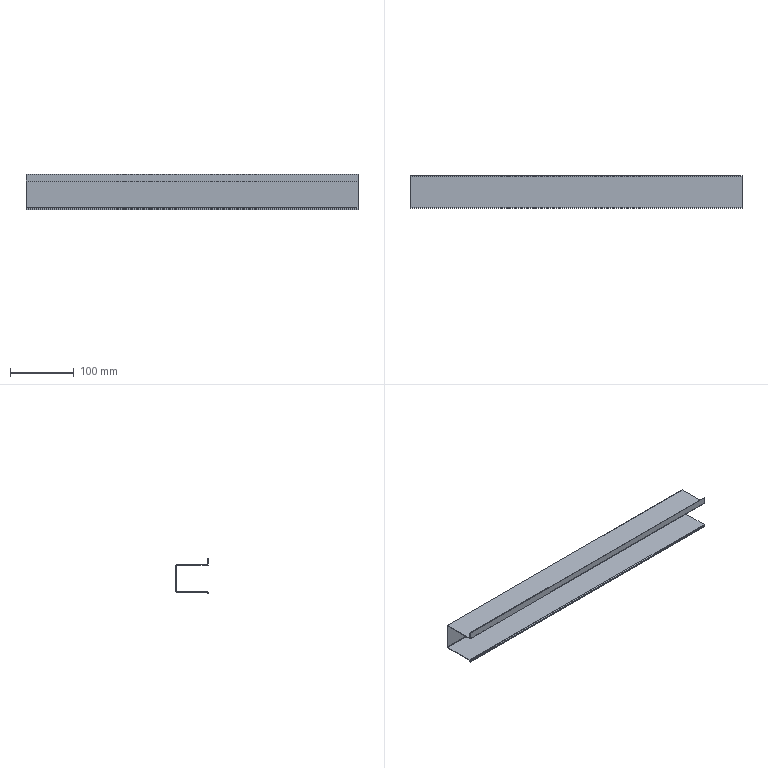Component | SolidWorks | ConnectingFlange-3 | 2 solids | 26 faces | box 520 x 50.74 x 55.53 mm | volume 58929 mm3 | plane 22 | cylinder 4 | commonest cylinder face diameters 2.946 x2 1.473 x2
STEP:
#1=COLOUR_RGB('',0.7922,0.8196,0.9333);
#2=FILL_AREA_STYLE_COLOUR('',#1);
#3=FILL_AREA_STYLE('',(#2));
#4=SURFACE_STYLE_FILL_AREA(#3);
#5=SURFACE_SIDE_STYLE('',(#4));
#6=SURFACE_STYLE_USAGE(.BOTH.,#5);
#7=PRESENTATION_STYLE_ASSIGNMENT((#6));
#8=CARTESIAN_POINT('',(-10.906,0.8454,1.916));
#9=VERTEX_POINT('',#8);
#10=CARTESIAN_POINT('',(-10.906,0.8454,1.945));
#11=VERTEX_POINT('',#10);
#12=CARTESIAN_POINT('',(-10.906,0.8454,1.916));
#13=DIRECTION('',(0.,-0.,1.));
#14=VECTOR('',#13,39.37);
#15=LINE('',#12,#14);
#16=EDGE_CURVE('',#9,#11,#15,.T.);
#17=ORIENTED_EDGE('',*,*,#16,.T.);
#18=CARTESIAN_POINT('',(-10.906,2.727,1.945));
#19=VERTEX_POINT('',#18);
#20=CARTESIAN_POINT('',(-10.906,2.756,1.945));
#21=DIRECTION('',(-0.,1.,0.));
#22=VECTOR('',#21,39.37);
#23=LINE('',#20,#22);
#24=EDGE_CURVE('',#11,#19,#23,.T.);
#25=ORIENTED_EDGE('',*,*,#24,.T.);
#26=CARTESIAN_POINT('',(-10.906,2.727,1.916));
#27=VERTEX_POINT('',#26);
#28=CARTESIAN_POINT('',(-10.906,2.727,1.916));
#29=DIRECTION('',(0.,0.,-1.));
#30=VECTOR('',#29,39.37);
#31=LINE('',#28,#30);
#32=EDGE_CURVE('',#19,#27,#31,.T.);
#33=ORIENTED_EDGE('',*,*,#32,.T.);
#34=CARTESIAN_POINT('',(-10.906,0.7874,1.916));
#35=DIRECTION('',(-0.,1.,0.));
#36=VECTOR('',#35,39.37);
#37=LINE('',#34,#36);
#38=EDGE_CURVE('',#9,#27,#37,.T.);
#39=ORIENTED_EDGE('',*,*,#38,.F.);
#40=EDGE_LOOP('',(#17,#25,#33,#39));
#41=FACE_OUTER_BOUND('',#40,.T.);
#42=CARTESIAN_POINT('',(-10.906,2.756,1.916));
#43=DIRECTION('',(1.,-0.,0.));
#44=DIRECTION('',(0.,0.,-1.));
#45=AXIS2_PLACEMENT_3D('',#42,#43,#44);
#46=PLANE('',#45);
#47=ADVANCED_FACE('',(#41),#46,.F.);
#48=CARTESIAN_POINT('',(9.567,2.727,1.916));
#49=VERTEX_POINT('',#48);
#50=CARTESIAN_POINT('',(-10.906,2.727,1.916));
#51=DIRECTION('',(-1.,0.,-0.));
#52=VECTOR('',#51,39.37);
#53=LINE('',#50,#52);
#54=EDGE_CURVE('',#49,#27,#53,.T.);
#55=ORIENTED_EDGE('',*,*,#54,.F.);
#56=CARTESIAN_POINT('',(9.567,0.8454,1.916));
#57=VERTEX_POINT('',#56);
#58=CARTESIAN_POINT('',(9.567,0.7874,1.916));
#59=DIRECTION('',(0.,-1.,-0.));
#60=VECTOR('',#59,39.37);
#61=LINE('',#58,#60);
#62=EDGE_CURVE('',#49,#57,#61,.T.);
#63=ORIENTED_EDGE('',*,*,#62,.T.);
#64=CARTESIAN_POINT('',(-10.906,0.8454,1.916));
#65=DIRECTION('',(1.,-0.,-0.));
#66=VECTOR('',#65,39.37);
#67=LINE('',#64,#66);
#68=EDGE_CURVE('',#9,#57,#67,.T.);
#69=ORIENTED_EDGE('',*,*,#68,.F.);
#70=ORIENTED_EDGE('',*,*,#38,.T.);
#71=EDGE_LOOP('',(#55,#63,#69,#70));
#72=FACE_OUTER_BOUND('',#71,.T.);
#73=CARTESIAN_POINT('',(0.,0.7874,1.916));
#74=DIRECTION('',(-0.,-0.,1.));
#75=DIRECTION('',(-0.,1.,0.));
#76=AXIS2_PLACEMENT_3D('',#73,#74,#75);
#77=PLANE('',#76);
#78=ADVANCED_FACE('',(#72),#77,.F.);
#79=CARTESIAN_POINT('',(9.567,2.727,1.945));
#80=VERTEX_POINT('',#79);
#81=CARTESIAN_POINT('',(9.567,0.8454,1.945));
#82=VERTEX_POINT('',#81);
#83=CARTESIAN_POINT('',(9.567,0.7874,1.945));
#84=DIRECTION('',(0.,-1.,-0.));
#85=VECTOR('',#84,39.37);
#86=LINE('',#83,#85);
#87=EDGE_CURVE('',#80,#82,#86,.T.);
#88=ORIENTED_EDGE('',*,*,#87,.F.);
#89=CARTESIAN_POINT('',(-10.906,2.727,1.945));
#90=DIRECTION('',(1.,-0.,0.));
#91=VECTOR('',#90,39.37);
#92=LINE('',#89,#91);
#93=EDGE_CURVE('',#19,#80,#92,.T.);
#94=ORIENTED_EDGE('',*,*,#93,.F.);
#95=ORIENTED_EDGE('',*,*,#24,.F.);
#96=CARTESIAN_POINT('',(-10.906,0.8454,1.945));
#97=DIRECTION('',(1.,-0.,-0.));
#98=VECTOR('',#97,39.37);
#99=LINE('',#96,#98);
#100=EDGE_CURVE('',#11,#82,#99,.T.);
#101=ORIENTED_EDGE('',*,*,#100,.T.);
#102=EDGE_LOOP('',(#88,#94,#95,#101));
#103=FACE_OUTER_BOUND('',#102,.T.);
#104=CARTESIAN_POINT('',(0.,0.7874,1.945));
#105=DIRECTION('',(-0.,-0.,1.));
#106=DIRECTION('',(-0.,1.,0.));
#107=AXIS2_PLACEMENT_3D('',#104,#105,#106);
#108=PLANE('',#107);
#109=ADVANCED_FACE('',(#103),#108,.T.);
#110=CARTESIAN_POINT('',(-10.906,2.785,3.579));
#111=VERTEX_POINT('',#110);
#112=CARTESIAN_POINT('',(9.567,2.785,3.579));
#113=VERTEX_POINT('',#112);
#114=CARTESIAN_POINT('',(-10.906,2.785,3.579));
#115=DIRECTION('',(1.,-0.,-0.));
#116=VECTOR('',#115,39.37);
#117=LINE('',#114,#116);
#118=EDGE_CURVE('',#111,#113,#117,.T.);
#119=ORIENTED_EDGE('',*,*,#118,.T.);
#120=CARTESIAN_POINT('',(9.567,2.785,1.974));
#121=VERTEX_POINT('',#120);
#122=CARTESIAN_POINT('',(9.567,2.785,-19.895));
#123=DIRECTION('',(-0.,0.,-1.));
#124=VECTOR('',#123,39.37);
#125=LINE('',#122,#124);
#126=EDGE_CURVE('',#113,#121,#125,.T.);
#127=ORIENTED_EDGE('',*,*,#126,.T.);
#128=CARTESIAN_POINT('',(-10.906,2.785,1.974));
#129=VERTEX_POINT('',#128);
#130=CARTESIAN_POINT('',(10.906,2.785,1.974));
#131=DIRECTION('',(-1.,0.,0.));
#132=VECTOR('',#131,39.37);
#133=LINE('',#130,#132);
#134=EDGE_CURVE('',#121,#129,#133,.T.);
#135=ORIENTED_EDGE('',*,*,#134,.T.);
#136=CARTESIAN_POINT('',(-10.906,2.785,-19.895));
#137=DIRECTION('',(0.,-0.,1.));
#138=VECTOR('',#137,39.37);
#139=LINE('',#136,#138);
#140=EDGE_CURVE('',#129,#111,#139,.T.);
#141=ORIENTED_EDGE('',*,*,#140,.T.);
#142=EDGE_LOOP('',(#119,#127,#135,#141));
#143=FACE_OUTER_BOUND('',#142,.T.);
#144=CARTESIAN_POINT('',(-10.906,2.785,-19.895));
#145=DIRECTION('',(-0.,-1.,-0.));
#146=DIRECTION('',(1.,-0.,-0.));
#147=AXIS2_PLACEMENT_3D('',#144,#145,#146);
#148=PLANE('',#147);
#149=ADVANCED_FACE('',(#143),#148,.F.);
#150=CARTESIAN_POINT('',(9.567,2.756,3.579));
#151=VERTEX_POINT('',#150);
#152=CARTESIAN_POINT('',(9.567,2.756,1.974));
#153=VERTEX_POINT('',#152);
#154=CARTESIAN_POINT('',(9.567,2.756,-19.895));
#155=DIRECTION('',(-0.,0.,-1.));
#156=VECTOR('',#155,39.37);
#157=LINE('',#154,#156);
#158=EDGE_CURVE('',#151,#153,#157,.T.);
#159=ORIENTED_EDGE('',*,*,#158,.F.);
#160=CARTESIAN_POINT('',(-10.906,2.756,3.579));
#161=VERTEX_POINT('',#160);
#162=CARTESIAN_POINT('',(-10.906,2.756,3.579));
#163=DIRECTION('',(1.,-0.,-0.));
#164=VECTOR('',#163,39.37);
#165=LINE('',#162,#164);
#166=EDGE_CURVE('',#161,#151,#165,.T.);
#167=ORIENTED_EDGE('',*,*,#166,.F.);
#168=CARTESIAN_POINT('',(-10.906,2.756,1.974));
#169=VERTEX_POINT('',#168);
#170=CARTESIAN_POINT('',(-10.906,2.756,-19.895));
#171=DIRECTION('',(0.,-0.,1.));
#172=VECTOR('',#171,39.37);
#173=LINE('',#170,#172);
#174=EDGE_CURVE('',#169,#161,#173,.T.);
#175=ORIENTED_EDGE('',*,*,#174,.F.);
#176=CARTESIAN_POINT('',(10.906,2.756,1.974));
#177=DIRECTION('',(-1.,0.,0.));
#178=VECTOR('',#177,39.37);
#179=LINE('',#176,#178);
#180=EDGE_CURVE('',#153,#169,#179,.T.);
#181=ORIENTED_EDGE('',*,*,#180,.F.);
#182=EDGE_LOOP('',(#159,#167,#175,#181));
#183=FACE_OUTER_BOUND('',#182,.T.);
#184=CARTESIAN_POINT('',(-10.906,2.756,-19.895));
#185=DIRECTION('',(-0.,-1.,-0.));
#186=DIRECTION('',(1.,-0.,-0.));
#187=AXIS2_PLACEMENT_3D('',#184,#185,#186);
#188=PLANE('',#187);
#189=ADVANCED_FACE('',(#183),#188,.T.);
#190=CARTESIAN_POINT('',(-10.906,2.756,1.974));
#191=DIRECTION('',(-0.,1.,0.));
#192=VECTOR('',#191,39.37);
#193=LINE('',#190,#192);
#194=EDGE_CURVE('',#169,#129,#193,.T.);
#195=ORIENTED_EDGE('',*,*,#194,.F.);
#196=ORIENTED_EDGE('',*,*,#174,.T.);
#197=CARTESIAN_POINT('',(-10.906,2.785,3.579));
#198=DIRECTION('',(0.,-1.,-0.));
#199=VECTOR('',#198,39.37);
#200=LINE('',#197,#199);
#201=EDGE_CURVE('',#111,#161,#200,.T.);
#202=ORIENTED_EDGE('',*,*,#201,.F.);
#203=ORIENTED_EDGE('',*,*,#140,.F.);
#204=EDGE_LOOP('',(#195,#196,#202,#203));
#205=FACE_OUTER_BOUND('',#204,.T.);
#206=CARTESIAN_POINT('',(-10.906,2.785,-19.895));
#207=DIRECTION('',(-1.,-0.,-0.));
#208=DIRECTION('',(0.,-1.,-0.));
#209=AXIS2_PLACEMENT_3D('',#206,#207,#208);
#210=PLANE('',#209);
#211=ADVANCED_FACE('',(#205),#210,.T.);
#212=ORIENTED_EDGE('',*,*,#166,.T.);
#213=CARTESIAN_POINT('',(9.567,0.7874,3.579));
#214=DIRECTION('',(-0.,1.,0.));
#215=VECTOR('',#214,39.37);
#216=LINE('',#213,#215);
#217=EDGE_CURVE('',#151,#113,#216,.T.);
#218=ORIENTED_EDGE('',*,*,#217,.T.);
#219=ORIENTED_EDGE('',*,*,#118,.F.);
#220=ORIENTED_EDGE('',*,*,#201,.T.);
#221=EDGE_LOOP('',(#212,#218,#219,#220));
#222=FACE_OUTER_BOUND('',#221,.T.);
#223=CARTESIAN_POINT('',(0.,0.7874,3.579));
#224=DIRECTION('',(0.,0.,-1.));
#225=DIRECTION('',(-1.,0.,0.));
#226=AXIS2_PLACEMENT_3D('',#223,#224,#225);
#227=PLANE('',#226);
#228=ADVANCED_FACE('',(#222),#227,.F.);
#229=ORIENTED_EDGE('',*,*,#32,.F.);
#230=CARTESIAN_POINT('',(-10.906,2.727,1.974));
#231=DIRECTION('',(-1.,0.,0.));
#232=DIRECTION('',(0.,1.,-0.));
#233=AXIS2_PLACEMENT_3D('',#230,#231,#232);
#234=CIRCLE('',#233,0.029);
#235=EDGE_CURVE('',#169,#19,#234,.T.);
#236=ORIENTED_EDGE('',*,*,#235,.F.);
#237=ORIENTED_EDGE('',*,*,#194,.T.);
#238=CARTESIAN_POINT('',(-10.906,2.727,1.974));
#239=DIRECTION('',(-1.,0.,0.));
#240=DIRECTION('',(0.,1.,0.));
#241=AXIS2_PLACEMENT_3D('',#238,#239,#240);
#242=CIRCLE('',#241,0.058);
#243=EDGE_CURVE('',#129,#27,#242,.T.);
#244=ORIENTED_EDGE('',*,*,#243,.T.);
#245=EDGE_LOOP('',(#229,#236,#237,#244));
#246=FACE_OUTER_BOUND('',#245,.T.);
#247=CARTESIAN_POINT('',(-10.906,2.727,1.974));
#248=DIRECTION('',(-1.,-0.,-0.));
#249=DIRECTION('',(0.,-1.,-0.));
#250=AXIS2_PLACEMENT_3D('',#247,#248,#249);
#251=PLANE('',#250);
#252=ADVANCED_FACE('',(#246),#251,.T.);
#253=CARTESIAN_POINT('',(9.567,2.727,1.974));
#254=DIRECTION('',(1.,-0.,-0.));
#255=DIRECTION('',(0.,-1.,0.));
#256=AXIS2_PLACEMENT_3D('',#253,#254,#255);
#257=CIRCLE('',#256,0.058);
#258=EDGE_CURVE('',#49,#121,#257,.T.);
#259=ORIENTED_EDGE('',*,*,#258,.F.);
#260=ORIENTED_EDGE('',*,*,#54,.T.);
#261=ORIENTED_EDGE('',*,*,#243,.F.);
#262=ORIENTED_EDGE('',*,*,#134,.F.);
#263=EDGE_LOOP('',(#259,#260,#261,#262));
#264=FACE_OUTER_BOUND('',#263,.T.);
#265=CARTESIAN_POINT('',(10.906,2.727,1.974));
#266=DIRECTION('',(1.,-0.,-0.));
#267=DIRECTION('',(0.,0.,-1.));
#268=AXIS2_PLACEMENT_3D('',#265,#266,#267);
#269=CYLINDRICAL_SURFACE('',#268,0.058);
#270=ADVANCED_FACE('',(#264),#269,.T.);
#271=ORIENTED_EDGE('',*,*,#93,.T.);
#272=CARTESIAN_POINT('',(9.567,2.727,1.974));
#273=DIRECTION('',(1.,-0.,-0.));
#274=DIRECTION('',(0.,-1.,0.));
#275=AXIS2_PLACEMENT_3D('',#272,#273,#274);
#276=CIRCLE('',#275,0.029);
#277=EDGE_CURVE('',#80,#153,#276,.T.);
#278=ORIENTED_EDGE('',*,*,#277,.T.);
#279=ORIENTED_EDGE('',*,*,#180,.T.);
#280=ORIENTED_EDGE('',*,*,#235,.T.);
#281=EDGE_LOOP('',(#271,#278,#279,#280));
#282=FACE_OUTER_BOUND('',#281,.T.);
#283=CARTESIAN_POINT('',(10.906,2.727,1.974));
#284=DIRECTION('',(1.,-0.,-0.));
#285=DIRECTION('',(0.,0.,-1.));
#286=AXIS2_PLACEMENT_3D('',#283,#284,#285);
#287=CYLINDRICAL_SURFACE('',#286,0.029);
#288=ADVANCED_FACE('',(#282),#287,.F.);
#289=CARTESIAN_POINT('',(-10.906,0.8164,1.887));
#290=VERTEX_POINT('',#289);
#291=CARTESIAN_POINT('',(-10.906,0.8454,1.887));
#292=DIRECTION('',(-1.,0.,0.));
#293=DIRECTION('',(0.,-1.,0.));
#294=AXIS2_PLACEMENT_3D('',#291,#292,#293);
#295=CIRCLE('',#294,0.029);
#296=EDGE_CURVE('',#290,#9,#295,.T.);
#297=ORIENTED_EDGE('',*,*,#296,.F.);
#298=CARTESIAN_POINT('',(-10.906,0.7874,1.887));
#299=VERTEX_POINT('',#298);
#300=CARTESIAN_POINT('',(-10.906,0.8164,1.887));
#301=DIRECTION('',(0.,-1.,0.));
#302=VECTOR('',#301,39.37);
#303=LINE('',#300,#302);
#304=EDGE_CURVE('',#290,#299,#303,.T.);
#305=ORIENTED_EDGE('',*,*,#304,.T.);
#306=CARTESIAN_POINT('',(-10.906,0.8454,1.887));
#307=DIRECTION('',(-1.,0.,0.));
#308=DIRECTION('',(0.,-1.,0.));
#309=AXIS2_PLACEMENT_3D('',#306,#307,#308);
#310=CIRCLE('',#309,0.058);
#311=EDGE_CURVE('',#299,#11,#310,.T.);
#312=ORIENTED_EDGE('',*,*,#311,.T.);
#313=ORIENTED_EDGE('',*,*,#16,.F.);
#314=EDGE_LOOP('',(#297,#305,#312,#313));
#315=FACE_OUTER_BOUND('',#314,.T.);
#316=CARTESIAN_POINT('',(-10.906,0.8454,1.887));
#317=DIRECTION('',(1.,-0.,-0.));
#318=DIRECTION('',(0.,1.,0.));
#319=AXIS2_PLACEMENT_3D('',#316,#317,#318);
#320=PLANE('',#319);
#321=ADVANCED_FACE('',(#315),#320,.F.);
#322=CARTESIAN_POINT('',(9.567,0.7874,1.887));
#323=VERTEX_POINT('',#322);
#324=CARTESIAN_POINT('',(9.567,0.8454,1.887));
#325=DIRECTION('',(1.,-0.,-0.));
#326=DIRECTION('',(0.,-1.,-0.));
#327=AXIS2_PLACEMENT_3D('',#324,#325,#326);
#328=CIRCLE('',#327,0.058);
#329=EDGE_CURVE('',#82,#323,#328,.T.);
#330=ORIENTED_EDGE('',*,*,#329,.F.);
#331=ORIENTED_EDGE('',*,*,#100,.F.);
#332=ORIENTED_EDGE('',*,*,#311,.F.);
#333=CARTESIAN_POINT('',(10.906,0.7874,1.887));
#334=DIRECTION('',(1.,-0.,0.));
#335=VECTOR('',#334,39.37);
#336=LINE('',#333,#335);
#337=EDGE_CURVE('',#299,#323,#336,.T.);
#338=ORIENTED_EDGE('',*,*,#337,.T.);
#339=EDGE_LOOP('',(#330,#331,#332,#338));
#340=FACE_OUTER_BOUND('',#339,.T.);
#341=CARTESIAN_POINT('',(-10.906,0.8454,1.887));
#342=DIRECTION('',(-1.,0.,0.));
#343=DIRECTION('',(0.,-1.,0.));
#344=AXIS2_PLACEMENT_3D('',#341,#342,#343);
#345=CYLINDRICAL_SURFACE('',#344,0.058);
#346=ADVANCED_FACE('',(#340),#345,.T.);
#347=ORIENTED_EDGE('',*,*,#68,.T.);
#348=CARTESIAN_POINT('',(9.567,0.8164,1.887));
#349=VERTEX_POINT('',#348);
#350=CARTESIAN_POINT('',(9.567,0.8454,1.887));
#351=DIRECTION('',(1.,-0.,-0.));
#352=DIRECTION('',(0.,-1.,-0.));
#353=AXIS2_PLACEMENT_3D('',#350,#351,#352);
#354=CIRCLE('',#353,0.029);
#355=EDGE_CURVE('',#57,#349,#354,.T.);
#356=ORIENTED_EDGE('',*,*,#355,.T.);
#357=CARTESIAN_POINT('',(10.906,0.8164,1.887));
#358=DIRECTION('',(-1.,0.,-0.));
#359=VECTOR('',#358,39.37);
#360=LINE('',#357,#359);
#361=EDGE_CURVE('',#349,#290,#360,.T.);
#362=ORIENTED_EDGE('',*,*,#361,.T.);
#363=ORIENTED_EDGE('',*,*,#296,.T.);
#364=EDGE_LOOP('',(#347,#356,#362,#363));
#365=FACE_OUTER_BOUND('',#364,.T.);
#366=CARTESIAN_POINT('',(-10.906,0.8454,1.887));
#367=DIRECTION('',(-1.,0.,0.));
#368=DIRECTION('',(0.,-1.,0.));
#369=AXIS2_PLACEMENT_3D('',#366,#367,#368);
#370=CYLINDRICAL_SURFACE('',#369,0.029);
#371=ADVANCED_FACE('',(#365),#370,.F.);
#372=ORIENTED_EDGE('',*,*,#304,.F.);
#373=CARTESIAN_POINT('',(-10.906,0.8164,1.815));
#374=VERTEX_POINT('',#373);
#375=CARTESIAN_POINT('',(-10.906,0.8164,1.815));
#376=DIRECTION('',(-0.,0.,-1.));
#377=VECTOR('',#376,39.37);
#378=LINE('',#375,#377);
#379=EDGE_CURVE('',#290,#374,#378,.T.);
#380=ORIENTED_EDGE('',*,*,#379,.T.);
#381=CARTESIAN_POINT('',(-10.906,0.7874,1.815));
#382=VERTEX_POINT('',#381);
#383=CARTESIAN_POINT('',(-10.906,0.7874,1.815));
#384=DIRECTION('',(-0.,1.,0.));
#385=VECTOR('',#384,39.37);
#386=LINE('',#383,#385);
#387=EDGE_CURVE('',#382,#374,#386,.T.);
#388=ORIENTED_EDGE('',*,*,#387,.F.);
#389=CARTESIAN_POINT('',(-10.906,0.7874,0.));
#390=DIRECTION('',(-0.,0.,-1.));
#391=VECTOR('',#390,39.37);
#392=LINE('',#389,#391);
#393=EDGE_CURVE('',#299,#382,#392,.T.);
#394=ORIENTED_EDGE('',*,*,#393,.F.);
#395=EDGE_LOOP('',(#372,#380,#388,#394));
#396=FACE_OUTER_BOUND('',#395,.T.);
#397=CARTESIAN_POINT('',(-10.906,0.7874,1.815));
#398=DIRECTION('',(1.,0.,0.));
#399=DIRECTION('',(-0.,1.,0.));
#400=AXIS2_PLACEMENT_3D('',#397,#398,#399);
#401=PLANE('',#400);
#402=ADVANCED_FACE('',(#396),#401,.F.);
#403=CARTESIAN_POINT('',(9.567,0.7874,1.815));
#404=VERTEX_POINT('',#403);
#405=CARTESIAN_POINT('',(0.,0.7874,1.815));
#406=DIRECTION('',(1.,-0.,0.));
#407=VECTOR('',#406,39.37);
#408=LINE('',#405,#407);
#409=EDGE_CURVE('',#382,#404,#408,.T.);
#410=ORIENTED_EDGE('',*,*,#409,.T.);
#411=CARTESIAN_POINT('',(9.567,0.7874,-4.553));
#412=DIRECTION('',(0.,-0.,1.));
#413=VECTOR('',#412,39.37);
#414=LINE('',#411,#413);
#415=EDGE_CURVE('',#404,#323,#414,.T.);
#416=ORIENTED_EDGE('',*,*,#415,.T.);
#417=ORIENTED_EDGE('',*,*,#337,.F.);
#418=ORIENTED_EDGE('',*,*,#393,.T.);
#419=EDGE_LOOP('',(#410,#416,#417,#418));
#420=FACE_OUTER_BOUND('',#419,.T.);
#421=CARTESIAN_POINT('',(0.,0.7874,0.));
#422=DIRECTION('',(-0.,1.,0.));
#423=DIRECTION('',(-0.,0.,-1.));
#424=AXIS2_PLACEMENT_3D('',#421,#422,#423);
#425=PLANE('',#424);
#426=ADVANCED_FACE('',(#420),#425,.F.);
#427=CARTESIAN_POINT('',(9.567,0.8164,1.815));
#428=VERTEX_POINT('',#427);
#429=CARTESIAN_POINT('',(9.567,0.8164,0.));
#430=DIRECTION('',(0.,-0.,1.));
#431=VECTOR('',#430,39.37);
#432=LINE('',#429,#431);
#433=EDGE_CURVE('',#428,#349,#432,.T.);
#434=ORIENTED_EDGE('',*,*,#433,.F.);
#435=CARTESIAN_POINT('',(10.906,0.8164,1.815));
#436=DIRECTION('',(1.,-0.,0.));
#437=VECTOR('',#436,39.37);
#438=LINE('',#435,#437);
#439=EDGE_CURVE('',#374,#428,#438,.T.);
#440=ORIENTED_EDGE('',*,*,#439,.F.);
#441=ORIENTED_EDGE('',*,*,#379,.F.);
#442=ORIENTED_EDGE('',*,*,#361,.F.);
#443=EDGE_LOOP('',(#434,#440,#441,#442));
#444=FACE_OUTER_BOUND('',#443,.T.);
#445=CARTESIAN_POINT('',(0.,0.8164,0.));
#446=DIRECTION('',(-0.,1.,0.));
#447=DIRECTION('',(-0.,0.,-1.));
#448=AXIS2_PLACEMENT_3D('',#445,#446,#447);
#449=PLANE('',#448);
#450=ADVANCED_FACE('',(#444),#449,.T.);
#451=ORIENTED_EDGE('',*,*,#439,.T.);
#452=CARTESIAN_POINT('',(9.567,0.7874,1.815));
#453=DIRECTION('',(0.,-1.,-0.));
#454=VECTOR('',#453,39.37);
#455=LINE('',#452,#454);
#456=EDGE_CURVE('',#428,#404,#455,.T.);
#457=ORIENTED_EDGE('',*,*,#456,.T.);
#458=ORIENTED_EDGE('',*,*,#409,.F.);
#459=ORIENTED_EDGE('',*,*,#387,.T.);
#460=EDGE_LOOP('',(#451,#457,#458,#459));
#461=FACE_OUTER_BOUND('',#460,.T.);
#462=CARTESIAN_POINT('',(10.906,0.7874,1.815));
#463=DIRECTION('',(-0.,-0.,1.));
#464=DIRECTION('',(1.,-0.,0.));
#465=AXIS2_PLACEMENT_3D('',#462,#463,#464);
#466=PLANE('',#465);
#467=ADVANCED_FACE('',(#461),#466,.F.);
#468=ORIENTED_EDGE('',*,*,#329,.T.);
#469=ORIENTED_EDGE('',*,*,#415,.F.);
#470=ORIENTED_EDGE('',*,*,#456,.F.);
#471=ORIENTED_EDGE('',*,*,#433,.T.);
#472=ORIENTED_EDGE('',*,*,#355,.F.);
#473=ORIENTED_EDGE('',*,*,#62,.F.);
#474=ORIENTED_EDGE('',*,*,#258,.T.);
#475=ORIENTED_EDGE('',*,*,#126,.F.);
#476=ORIENTED_EDGE('',*,*,#217,.F.);
#477=ORIENTED_EDGE('',*,*,#158,.T.);
#478=ORIENTED_EDGE('',*,*,#277,.F.);
#479=ORIENTED_EDGE('',*,*,#87,.T.);
#480=EDGE_LOOP('',(#468,#469,#470,#471,#472,#473,#474,#475,#476,#477,#478,#479));
#481=FACE_OUTER_BOUND('',#480,.T.);
#482=CARTESIAN_POINT('',(9.567,0.7874,-4.553));
#483=DIRECTION('',(-1.,-0.,-0.));
#484=DIRECTION('',(0.,-1.,-0.));
#485=AXIS2_PLACEMENT_3D('',#482,#483,#484);
#486=PLANE('',#485);
#487=ADVANCED_FACE('',(#481),#486,.F.);
#488=CLOSED_SHELL('',(#47,#78,#109,#149,#189,#211,#228,#252,#270,#288,#321,#346,#371,#402,#426,#450,#467,#487));
#489=MANIFOLD_SOLID_BREP('',#488);
#490=STYLED_ITEM('',(#7),#489);
#491=(LENGTH_UNIT()NAMED_UNIT(*)SI_UNIT($,.METRE.));
#492=LENGTH_MEASURE_WITH_UNIT(LENGTH_MEASURE(0.0254),#491);
#493=DIMENSIONAL_EXPONENTS(1.,0.,0.,0.,0.,0.,0.);
#494=(CONVERSION_BASED_UNIT('',#492)LENGTH_UNIT()NAMED_UNIT(#493));
#495=UNCERTAINTY_MEASURE_WITH_UNIT(LENGTH_MEASURE(0.00001),#494,'','');
#496=(NAMED_UNIT(*)PLANE_ANGLE_UNIT()SI_UNIT($,.RADIAN.));
#497=(NAMED_UNIT(*)SI_UNIT($,.STERADIAN.)SOLID_ANGLE_UNIT());
#498=(GEOMETRIC_REPRESENTATION_CONTEXT(3)GLOBAL_UNCERTAINTY_ASSIGNED_CONTEXT((#495))GLOBAL_UNIT_ASSIGNED_CONTEXT((#494,#496,#497))REPRESENTATION_CONTEXT('',''));
#499=MECHANICAL_DESIGN_GEOMETRIC_PRESENTATION_REPRESENTATION('',(#490),#498);
#500=COLOUR_RGB('',0.7922,0.8196,0.9333);
#501=FILL_AREA_STYLE_COLOUR('',#500);
#502=FILL_AREA_STYLE('',(#501));
#503=SURFACE_STYLE_FILL_AREA(#502);
#504=SURFACE_SIDE_STYLE('',(#503));
#505=SURFACE_STYLE_USAGE(.BOTH.,#504);
#506=PRESENTATION_STYLE_ASSIGNMENT((#505));
#507=CARTESIAN_POINT('',(9.567,0.8164,3.608));
#508=VERTEX_POINT('',#507);
#509=CARTESIAN_POINT('',(-10.906,0.8164,3.608));
#510=VERTEX_POINT('',#509);
#511=CARTESIAN_POINT('',(10.906,0.8164,3.608));
#512=DIRECTION('',(-1.,0.,0.));
#513=VECTOR('',#512,39.37);
#514=LINE('',#511,#513);
#515=EDGE_CURVE('',#508,#510,#514,.T.);
#516=ORIENTED_EDGE('',*,*,#515,.F.);
#517=CARTESIAN_POINT('',(9.567,2.756,3.608));
#518=VERTEX_POINT('',#517);
#519=CARTESIAN_POINT('',(9.567,2.756,3.608));
#520=DIRECTION('',(-0.,1.,0.));
#521=VECTOR('',#520,39.37);
#522=LINE('',#519,#521);
#523=EDGE_CURVE('',#508,#518,#522,.T.);
#524=ORIENTED_EDGE('',*,*,#523,.T.);
#525=CARTESIAN_POINT('',(-10.906,2.756,3.608));
#526=VERTEX_POINT('',#525);
#527=CARTESIAN_POINT('',(-10.906,2.756,3.608));
#528=DIRECTION('',(1.,-0.,-0.));
#529=VECTOR('',#528,39.37);
#530=LINE('',#527,#529);
#531=EDGE_CURVE('',#526,#518,#530,.T.);
#532=ORIENTED_EDGE('',*,*,#531,.F.);
#533=CARTESIAN_POINT('',(-10.906,2.756,3.608));
#534=DIRECTION('',(0.,-1.,-0.));
#535=VECTOR('',#534,39.37);
#536=LINE('',#533,#535);
#537=EDGE_CURVE('',#526,#510,#536,.T.);
#538=ORIENTED_EDGE('',*,*,#537,.T.);
#539=EDGE_LOOP('',(#516,#524,#532,#538));
#540=FACE_OUTER_BOUND('',#539,.T.);
#541=CARTESIAN_POINT('',(-10.906,2.756,3.608));
#542=DIRECTION('',(-0.,0.,-1.));
#543=DIRECTION('',(0.,-1.,-0.));
#544=AXIS2_PLACEMENT_3D('',#541,#542,#543);
#545=PLANE('',#544);
#546=ADVANCED_FACE('',(#540),#545,.F.);
#547=CARTESIAN_POINT('',(9.567,0.7874,3.579));
#548=VERTEX_POINT('',#547);
#549=CARTESIAN_POINT('',(9.567,2.756,3.579));
#550=VERTEX_POINT('',#549);
#551=CARTESIAN_POINT('',(9.567,2.756,3.579));
#552=DIRECTION('',(-0.,1.,0.));
#553=VECTOR('',#552,39.37);
#554=LINE('',#551,#553);
#555=EDGE_CURVE('',#548,#550,#554,.T.);
#556=ORIENTED_EDGE('',*,*,#555,.F.);
#557=CARTESIAN_POINT('',(-10.906,0.7874,3.579));
#558=VERTEX_POINT('',#557);
#559=CARTESIAN_POINT('',(-10.906,0.7874,3.579));
#560=DIRECTION('',(1.,-0.,-0.));
#561=VECTOR('',#560,39.37);
#562=LINE('',#559,#561);
#563=EDGE_CURVE('',#558,#548,#562,.T.);
#564=ORIENTED_EDGE('',*,*,#563,.F.);
#565=CARTESIAN_POINT('',(-10.906,2.756,3.579));
#566=VERTEX_POINT('',#565);
#567=CARTESIAN_POINT('',(-10.906,2.756,3.579));
#568=DIRECTION('',(0.,-1.,-0.));
#569=VECTOR('',#568,39.37);
#570=LINE('',#567,#569);
#571=EDGE_CURVE('',#566,#558,#570,.T.);
#572=ORIENTED_EDGE('',*,*,#571,.F.);
#573=CARTESIAN_POINT('',(-10.906,2.756,3.579));
#574=DIRECTION('',(1.,-0.,-0.));
#575=VECTOR('',#574,39.37);
#576=LINE('',#573,#575);
#577=EDGE_CURVE('',#566,#550,#576,.T.);
#578=ORIENTED_EDGE('',*,*,#577,.T.);
#579=EDGE_LOOP('',(#556,#564,#572,#578));
#580=FACE_OUTER_BOUND('',#579,.T.);
#581=CARTESIAN_POINT('',(-10.906,2.756,3.579));
#582=DIRECTION('',(-0.,0.,-1.));
#583=DIRECTION('',(0.,-1.,-0.));
#584=AXIS2_PLACEMENT_3D('',#581,#582,#583);
#585=PLANE('',#584);
#586=ADVANCED_FACE('',(#580),#585,.T.);
#587=CARTESIAN_POINT('',(-10.906,0.7874,4.001));
#588=VERTEX_POINT('',#587);
#589=CARTESIAN_POINT('',(-10.906,0.7874,3.608));
#590=DIRECTION('',(-0.,0.,-1.));
#591=VECTOR('',#590,39.37);
#592=LINE('',#589,#591);
#593=EDGE_CURVE('',#588,#558,#592,.T.);
#594=ORIENTED_EDGE('',*,*,#593,.F.);
#595=CARTESIAN_POINT('',(-10.906,0.8164,4.001));
#596=VERTEX_POINT('',#595);
#597=CARTESIAN_POINT('',(-10.906,0.7874,4.001));
#598=DIRECTION('',(-0.,1.,0.));
#599=VECTOR('',#598,39.37);
#600=LINE('',#597,#599);
#601=EDGE_CURVE('',#588,#596,#600,.T.);
#602=ORIENTED_EDGE('',*,*,#601,.T.);
#603=CARTESIAN_POINT('',(-10.906,0.8164,4.001));
#604=DIRECTION('',(-0.,0.,-1.));
#605=VECTOR('',#604,39.37);
#606=LINE('',#603,#605);
#607=EDGE_CURVE('',#596,#510,#606,.T.);
#608=ORIENTED_EDGE('',*,*,#607,.T.);
#609=ORIENTED_EDGE('',*,*,#537,.F.);
#610=CARTESIAN_POINT('',(-10.906,2.756,3.608));
#611=DIRECTION('',(-0.,0.,-1.));
#612=VECTOR('',#611,39.37);
#613=LINE('',#610,#612);
#614=EDGE_CURVE('',#526,#566,#613,.T.);
#615=ORIENTED_EDGE('',*,*,#614,.T.);
#616=ORIENTED_EDGE('',*,*,#571,.T.);
#617=EDGE_LOOP('',(#594,#602,#608,#609,#615,#616));
#618=FACE_OUTER_BOUND('',#617,.T.);
#619=CARTESIAN_POINT('',(-10.906,2.756,3.608));
#620=DIRECTION('',(-1.,-0.,-0.));
#621=DIRECTION('',(0.,-1.,-0.));
#622=AXIS2_PLACEMENT_3D('',#619,#620,#621);
#623=PLANE('',#622);
#624=ADVANCED_FACE('',(#618),#623,.T.);
#625=CARTESIAN_POINT('',(9.567,2.756,0.));
#626=DIRECTION('',(0.,-0.,1.));
#627=VECTOR('',#626,39.37);
#628=LINE('',#625,#627);
#629=EDGE_CURVE('',#550,#518,#628,.T.);
#630=ORIENTED_EDGE('',*,*,#629,.F.);
#631=ORIENTED_EDGE('',*,*,#577,.F.);
#632=ORIENTED_EDGE('',*,*,#614,.F.);
#633=ORIENTED_EDGE('',*,*,#531,.T.);
#634=EDGE_LOOP('',(#630,#631,#632,#633));
#635=FACE_OUTER_BOUND('',#634,.T.);
#636=CARTESIAN_POINT('',(0.,2.756,0.));
#637=DIRECTION('',(0.,1.,0.));
#638=DIRECTION('',(-1.,0.,0.));
#639=AXIS2_PLACEMENT_3D('',#636,#637,#638);
#640=PLANE('',#639);
#641=ADVANCED_FACE('',(#635),#640,.T.);
#642=ORIENTED_EDGE('',*,*,#563,.T.);
#643=CARTESIAN_POINT('',(9.567,0.7874,4.001));
#644=VERTEX_POINT('',#643);
#645=CARTESIAN_POINT('',(9.567,0.7874,-4.553));
#646=DIRECTION('',(0.,-0.,1.));
#647=VECTOR('',#646,39.37);
#648=LINE('',#645,#647);
#649=EDGE_CURVE('',#548,#644,#648,.T.);
#650=ORIENTED_EDGE('',*,*,#649,.T.);
#651=CARTESIAN_POINT('',(10.906,0.7874,4.001));
#652=DIRECTION('',(-1.,0.,0.));
#653=VECTOR('',#652,39.37);
#654=LINE('',#651,#653);
#655=EDGE_CURVE('',#644,#588,#654,.T.);
#656=ORIENTED_EDGE('',*,*,#655,.T.);
#657=ORIENTED_EDGE('',*,*,#593,.T.);
#658=EDGE_LOOP('',(#642,#650,#656,#657));
#659=FACE_OUTER_BOUND('',#658,.T.);
#660=CARTESIAN_POINT('',(0.,0.7874,0.));
#661=DIRECTION('',(0.,1.,0.));
#662=DIRECTION('',(-1.,0.,0.));
#663=AXIS2_PLACEMENT_3D('',#660,#661,#662);
#664=PLANE('',#663);
#665=ADVANCED_FACE('',(#659),#664,.F.);
#666=CARTESIAN_POINT('',(9.567,0.8164,4.001));
#667=VERTEX_POINT('',#666);
#668=CARTESIAN_POINT('',(10.906,0.8164,4.001));
#669=DIRECTION('',(-1.,0.,0.));
#670=VECTOR('',#669,39.37);
#671=LINE('',#668,#670);
#672=EDGE_CURVE('',#667,#596,#671,.T.);
#673=ORIENTED_EDGE('',*,*,#672,.F.);
#674=CARTESIAN_POINT('',(9.567,0.8164,4.001));
#675=DIRECTION('',(-0.,0.,-1.));
#676=VECTOR('',#675,39.37);
#677=LINE('',#674,#676);
#678=EDGE_CURVE('',#667,#508,#677,.T.);
#679=ORIENTED_EDGE('',*,*,#678,.T.);
#680=ORIENTED_EDGE('',*,*,#515,.T.);
#681=ORIENTED_EDGE('',*,*,#607,.F.);
#682=EDGE_LOOP('',(#673,#679,#680,#681));
#683=FACE_OUTER_BOUND('',#682,.T.);
#684=CARTESIAN_POINT('',(10.906,0.8164,4.001));
#685=DIRECTION('',(-0.,-1.,-0.));
#686=DIRECTION('',(1.,-0.,-0.));
#687=AXIS2_PLACEMENT_3D('',#684,#685,#686);
#688=PLANE('',#687);
#689=ADVANCED_FACE('',(#683),#688,.F.);
#690=ORIENTED_EDGE('',*,*,#655,.F.);
#691=CARTESIAN_POINT('',(9.567,0.7874,4.001));
#692=DIRECTION('',(-0.,1.,0.));
#693=VECTOR('',#692,39.37);
#694=LINE('',#691,#693);
#695=EDGE_CURVE('',#644,#667,#694,.T.);
#696=ORIENTED_EDGE('',*,*,#695,.T.);
#697=ORIENTED_EDGE('',*,*,#672,.T.);
#698=ORIENTED_EDGE('',*,*,#601,.F.);
#699=EDGE_LOOP('',(#690,#696,#697,#698));
#700=FACE_OUTER_BOUND('',#699,.T.);
#701=CARTESIAN_POINT('',(0.,0.7874,4.001));
#702=DIRECTION('',(0.,0.,-1.));
#703=DIRECTION('',(1.,-0.,-0.));
#704=AXIS2_PLACEMENT_3D('',#701,#702,#703);
#705=PLANE('',#704);
#706=ADVANCED_FACE('',(#700),#705,.F.);
#707=ORIENTED_EDGE('',*,*,#555,.T.);
#708=ORIENTED_EDGE('',*,*,#629,.T.);
#709=ORIENTED_EDGE('',*,*,#523,.F.);
#710=ORIENTED_EDGE('',*,*,#678,.F.);
#711=ORIENTED_EDGE('',*,*,#695,.F.);
#712=ORIENTED_EDGE('',*,*,#649,.F.);
#713=EDGE_LOOP('',(#707,#708,#709,#710,#711,#712));
#714=FACE_OUTER_BOUND('',#713,.T.);
#715=CARTESIAN_POINT('',(9.567,0.7874,-4.553));
#716=DIRECTION('',(-1.,-0.,-0.));
#717=DIRECTION('',(0.,-1.,-0.));
#718=AXIS2_PLACEMENT_3D('',#715,#716,#717);
#719=PLANE('',#718);
#720=ADVANCED_FACE('',(#714),#719,.F.);
#721=CLOSED_SHELL('',(#546,#586,#624,#641,#665,#689,#706,#720));
#722=MANIFOLD_SOLID_BREP('',#721);
#723=STYLED_ITEM('',(#506),#722);
#724=PRESENTATION_LAYER_ASSIGNMENT('','',(#723));
#725=PRESENTATION_LAYER_ASSIGNMENT('','',(#490));
#726=CARTESIAN_POINT('',(0.,0.,0.));
#727=DIRECTION('',(0.,0.,1.));
#728=DIRECTION('',(1.,0.,0.));
#729=AXIS2_PLACEMENT_3D('',#726,#727,#728);
#730=(LENGTH_UNIT()NAMED_UNIT(*)SI_UNIT($,.METRE.));
#731=LENGTH_MEASURE_WITH_UNIT(LENGTH_MEASURE(0.0254),#730);
#732=DIMENSIONAL_EXPONENTS(1.,0.,0.,0.,0.,0.,0.);
#733=(CONVERSION_BASED_UNIT('',#731)LENGTH_UNIT()NAMED_UNIT(#732));
#734=UNCERTAINTY_MEASURE_WITH_UNIT(LENGTH_MEASURE(0.00001),#733,'','');
#735=(NAMED_UNIT(*)PLANE_ANGLE_UNIT()SI_UNIT($,.RADIAN.));
#736=(NAMED_UNIT(*)SI_UNIT($,.STERADIAN.)SOLID_ANGLE_UNIT());
#737=(GEOMETRIC_REPRESENTATION_CONTEXT(3)GLOBAL_UNCERTAINTY_ASSIGNED_CONTEXT((#734))GLOBAL_UNIT_ASSIGNED_CONTEXT((#733,#735,#736))REPRESENTATION_CONTEXT('',''));
#738=ADVANCED_BREP_SHAPE_REPRESENTATION('',(#489,#722,#729),#737);
#739=(LENGTH_UNIT()NAMED_UNIT(*)SI_UNIT($,.METRE.));
#740=LENGTH_MEASURE_WITH_UNIT(LENGTH_MEASURE(0.0254),#739);
#741=DIMENSIONAL_EXPONENTS(1.,0.,0.,0.,0.,0.,0.);
#742=(CONVERSION_BASED_UNIT('',#740)LENGTH_UNIT()NAMED_UNIT(#741));
#743=UNCERTAINTY_MEASURE_WITH_UNIT(LENGTH_MEASURE(0.00001),#742,'','');
#744=(NAMED_UNIT(*)PLANE_ANGLE_UNIT()SI_UNIT($,.RADIAN.));
#745=(NAMED_UNIT(*)SI_UNIT($,.STERADIAN.)SOLID_ANGLE_UNIT());
#746=(GEOMETRIC_REPRESENTATION_CONTEXT(3)GLOBAL_UNCERTAINTY_ASSIGNED_CONTEXT((#743))GLOBAL_UNIT_ASSIGNED_CONTEXT((#742,#744,#745))REPRESENTATION_CONTEXT('',''));
#747=MECHANICAL_DESIGN_GEOMETRIC_PRESENTATION_REPRESENTATION('',(#723),#746);